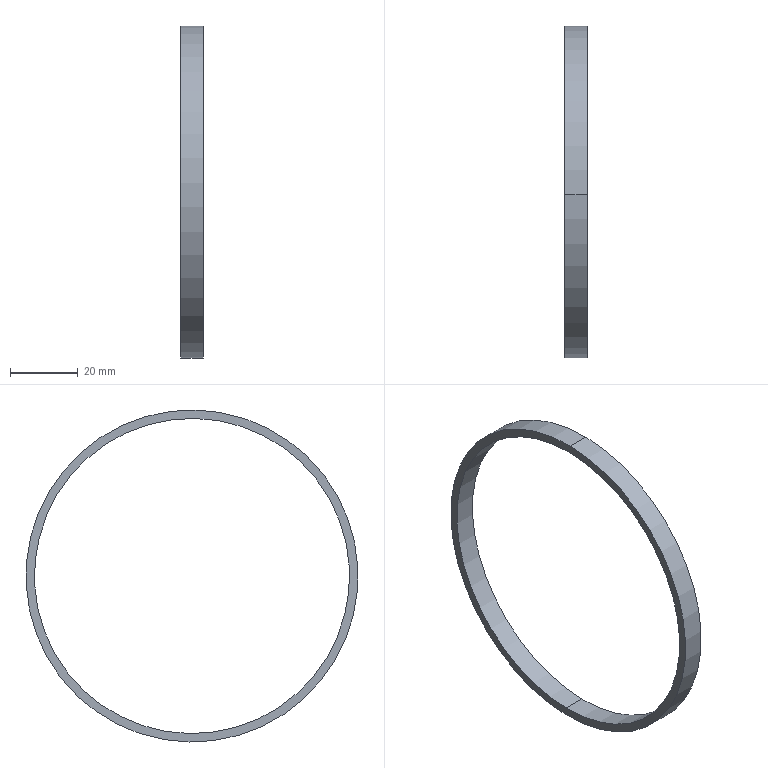Component | SolidWorks | 216InnerTubeAssembly-1_RetainingRing-1 | 1 solid | 6 faces | box 6.5 x 98 x 98 mm | volume 4875 mm3 | cylinder 4 | plane 2 | commonest cylinder face diameters 98 x2 93 x2 | material Alloy Steel
build123d program:
from build123d import *

# Parameters (mm, degrees)
MODEL_W = 6.5
MODEL_H = 2.5


with BuildPart() as part:
    # Model → Revolve1 (revolve)
    with BuildSketch(Plane.XY, mode=Mode.PRIVATE) as revolve1_sk:
        with Locations((3.25, 47.75)):
            Rectangle(MODEL_W, MODEL_H)
    revolve(revolve1_sk.sketch.rotate(Axis((0, 0, 0), (1, 0, 0)), 90), axis=Axis((0, 0, 0), (1, 0, 0)))


solid = part.part

# Placed as in the assembly
solid = solid.moved(Location((2893.278, 0, 0), (0, 0, 0)))
STEP:
#1=CARTESIAN_POINT('',(114.164,-0.03464,1.929));
#2=VERTEX_POINT('',#1);
#3=CARTESIAN_POINT('',(114.164,0.03464,-1.929));
#4=VERTEX_POINT('',#3);
#5=CARTESIAN_POINT('',(114.164,-0.,0.));
#6=DIRECTION('',(-1.,-0.,0.));
#7=DIRECTION('',(0.,-0.01796,0.9998));
#8=AXIS2_PLACEMENT_3D('',#5,#6,#7);
#9=CIRCLE('',#8,1.929);
#10=EDGE_CURVE('',#2,#4,#9,.T.);
#11=ORIENTED_EDGE('',*,*,#10,.T.);
#12=CARTESIAN_POINT('',(113.909,0.03464,-1.929));
#13=VERTEX_POINT('',#12);
#14=CARTESIAN_POINT('',(113.909,0.03464,-1.929));
#15=DIRECTION('',(-1.,-0.,0.));
#16=VECTOR('',#15,39.37);
#17=LINE('',#14,#16);
#18=EDGE_CURVE('',#4,#13,#17,.T.);
#19=ORIENTED_EDGE('',*,*,#18,.T.);
#20=CARTESIAN_POINT('',(113.909,-0.03464,1.929));
#21=VERTEX_POINT('',#20);
#22=CARTESIAN_POINT('',(113.909,-0.,0.));
#23=DIRECTION('',(-1.,-0.,0.));
#24=DIRECTION('',(0.,-0.01796,0.9998));
#25=AXIS2_PLACEMENT_3D('',#22,#23,#24);
#26=CIRCLE('',#25,1.929);
#27=EDGE_CURVE('',#21,#13,#26,.T.);
#28=ORIENTED_EDGE('',*,*,#27,.F.);
#29=CARTESIAN_POINT('',(113.909,-0.03464,1.929));
#30=DIRECTION('',(-1.,-0.,0.));
#31=VECTOR('',#30,39.37);
#32=LINE('',#29,#31);
#33=EDGE_CURVE('',#2,#21,#32,.T.);
#34=ORIENTED_EDGE('',*,*,#33,.F.);
#35=EDGE_LOOP('',(#11,#19,#28,#34));
#36=FACE_OUTER_BOUND('',#35,.T.);
#37=CARTESIAN_POINT('',(113.909,-0.,0.));
#38=DIRECTION('',(-1.,-0.,0.));
#39=DIRECTION('',(0.,-0.01796,0.9998));
#40=AXIS2_PLACEMENT_3D('',#37,#38,#39);
#41=CYLINDRICAL_SURFACE('',#40,1.929);
#42=ADVANCED_FACE('',(#36),#41,.T.);
#43=CARTESIAN_POINT('',(114.164,0.03287,-1.83));
#44=VERTEX_POINT('',#43);
#45=CARTESIAN_POINT('',(114.164,-0.03287,1.83));
#46=VERTEX_POINT('',#45);
#47=CARTESIAN_POINT('',(114.164,-0.,0.));
#48=DIRECTION('',(-1.,-0.,0.));
#49=DIRECTION('',(0.,-0.01796,0.9998));
#50=AXIS2_PLACEMENT_3D('',#47,#48,#49);
#51=CIRCLE('',#50,1.831);
#52=EDGE_CURVE('',#44,#46,#51,.T.);
#53=ORIENTED_EDGE('',*,*,#52,.F.);
#54=CARTESIAN_POINT('',(113.909,0.03287,-1.83));
#55=VERTEX_POINT('',#54);
#56=CARTESIAN_POINT('',(113.909,0.03287,-1.83));
#57=DIRECTION('',(-1.,-0.,0.));
#58=VECTOR('',#57,39.37);
#59=LINE('',#56,#58);
#60=EDGE_CURVE('',#44,#55,#59,.T.);
#61=ORIENTED_EDGE('',*,*,#60,.T.);
#62=CARTESIAN_POINT('',(113.909,-0.03287,1.83));
#63=VERTEX_POINT('',#62);
#64=CARTESIAN_POINT('',(113.909,-0.,0.));
#65=DIRECTION('',(-1.,-0.,0.));
#66=DIRECTION('',(0.,-0.01796,0.9998));
#67=AXIS2_PLACEMENT_3D('',#64,#65,#66);
#68=CIRCLE('',#67,1.831);
#69=EDGE_CURVE('',#55,#63,#68,.T.);
#70=ORIENTED_EDGE('',*,*,#69,.T.);
#71=CARTESIAN_POINT('',(113.909,-0.03287,1.83));
#72=DIRECTION('',(-1.,-0.,0.));
#73=VECTOR('',#72,39.37);
#74=LINE('',#71,#73);
#75=EDGE_CURVE('',#46,#63,#74,.T.);
#76=ORIENTED_EDGE('',*,*,#75,.F.);
#77=EDGE_LOOP('',(#53,#61,#70,#76));
#78=FACE_OUTER_BOUND('',#77,.T.);
#79=CARTESIAN_POINT('',(113.909,-0.,0.));
#80=DIRECTION('',(-1.,-0.,0.));
#81=DIRECTION('',(0.,-0.01796,0.9998));
#82=AXIS2_PLACEMENT_3D('',#79,#80,#81);
#83=CYLINDRICAL_SURFACE('',#82,1.831);
#84=ADVANCED_FACE('',(#78),#83,.F.);
#85=ORIENTED_EDGE('',*,*,#10,.F.);
#86=CARTESIAN_POINT('',(114.164,-0.,0.));
#87=DIRECTION('',(-1.,-0.,0.));
#88=DIRECTION('',(0.,-0.01796,0.9998));
#89=AXIS2_PLACEMENT_3D('',#86,#87,#88);
#90=CIRCLE('',#89,1.929);
#91=EDGE_CURVE('',#4,#2,#90,.T.);
#92=ORIENTED_EDGE('',*,*,#91,.F.);
#93=EDGE_LOOP('',(#85,#92));
#94=FACE_OUTER_BOUND('',#93,.T.);
#95=CARTESIAN_POINT('',(114.164,-0.,0.));
#96=DIRECTION('',(-1.,-0.,0.));
#97=DIRECTION('',(0.,-0.01796,0.9998));
#98=AXIS2_PLACEMENT_3D('',#95,#96,#97);
#99=CIRCLE('',#98,1.831);
#100=EDGE_CURVE('',#46,#44,#99,.T.);
#101=ORIENTED_EDGE('',*,*,#100,.T.);
#102=ORIENTED_EDGE('',*,*,#52,.T.);
#103=EDGE_LOOP('',(#101,#102));
#104=FACE_BOUND('',#103,.T.);
#105=CARTESIAN_POINT('',(114.164,1.929,0.03464));
#106=DIRECTION('',(-1.,-0.,0.));
#107=DIRECTION('',(0.,-0.01796,0.9998));
#108=AXIS2_PLACEMENT_3D('',#105,#106,#107);
#109=PLANE('',#108);
#110=ADVANCED_FACE('',(#94,#104),#109,.F.);
#111=ORIENTED_EDGE('',*,*,#60,.F.);
#112=ORIENTED_EDGE('',*,*,#100,.F.);
#113=ORIENTED_EDGE('',*,*,#75,.T.);
#114=CARTESIAN_POINT('',(113.909,-0.,0.));
#115=DIRECTION('',(-1.,-0.,0.));
#116=DIRECTION('',(0.,-0.01796,0.9998));
#117=AXIS2_PLACEMENT_3D('',#114,#115,#116);
#118=CIRCLE('',#117,1.831);
#119=EDGE_CURVE('',#63,#55,#118,.T.);
#120=ORIENTED_EDGE('',*,*,#119,.T.);
#121=EDGE_LOOP('',(#111,#112,#113,#120));
#122=FACE_OUTER_BOUND('',#121,.T.);
#123=CARTESIAN_POINT('',(113.909,-0.,0.));
#124=DIRECTION('',(-1.,-0.,0.));
#125=DIRECTION('',(0.,-0.01796,0.9998));
#126=AXIS2_PLACEMENT_3D('',#123,#124,#125);
#127=CYLINDRICAL_SURFACE('',#126,1.831);
#128=ADVANCED_FACE('',(#122),#127,.F.);
#129=ORIENTED_EDGE('',*,*,#119,.F.);
#130=ORIENTED_EDGE('',*,*,#69,.F.);
#131=EDGE_LOOP('',(#129,#130));
#132=FACE_BOUND('',#131,.T.);
#133=ORIENTED_EDGE('',*,*,#27,.T.);
#134=CARTESIAN_POINT('',(113.909,-0.,0.));
#135=DIRECTION('',(-1.,-0.,0.));
#136=DIRECTION('',(0.,-0.01796,0.9998));
#137=AXIS2_PLACEMENT_3D('',#134,#135,#136);
#138=CIRCLE('',#137,1.929);
#139=EDGE_CURVE('',#13,#21,#138,.T.);
#140=ORIENTED_EDGE('',*,*,#139,.T.);
#141=EDGE_LOOP('',(#133,#140));
#142=FACE_OUTER_BOUND('',#141,.T.);
#143=CARTESIAN_POINT('',(113.909,1.929,0.03464));
#144=DIRECTION('',(1.,0.,-0.));
#145=DIRECTION('',(-0.,0.01796,-0.9998));
#146=AXIS2_PLACEMENT_3D('',#143,#144,#145);
#147=PLANE('',#146);
#148=ADVANCED_FACE('',(#132,#142),#147,.F.);
#149=ORIENTED_EDGE('',*,*,#18,.F.);
#150=ORIENTED_EDGE('',*,*,#91,.T.);
#151=ORIENTED_EDGE('',*,*,#33,.T.);
#152=ORIENTED_EDGE('',*,*,#139,.F.);
#153=EDGE_LOOP('',(#149,#150,#151,#152));
#154=FACE_OUTER_BOUND('',#153,.T.);
#155=CARTESIAN_POINT('',(113.909,-0.,0.));
#156=DIRECTION('',(-1.,-0.,0.));
#157=DIRECTION('',(0.,-0.01796,0.9998));
#158=AXIS2_PLACEMENT_3D('',#155,#156,#157);
#159=CYLINDRICAL_SURFACE('',#158,1.929);
#160=ADVANCED_FACE('',(#154),#159,.T.);
#161=CLOSED_SHELL('',(#42,#84,#110,#128,#148,#160));
#162=MANIFOLD_SOLID_BREP('',#161);
#163=CARTESIAN_POINT('',(0.,0.,0.));
#164=DIRECTION('',(0.,0.,1.));
#165=DIRECTION('',(1.,0.,0.));
#166=AXIS2_PLACEMENT_3D('',#163,#164,#165);
#167=(LENGTH_UNIT()NAMED_UNIT(*)SI_UNIT($,.METRE.));
#168=LENGTH_MEASURE_WITH_UNIT(LENGTH_MEASURE(0.0254),#167);
#169=DIMENSIONAL_EXPONENTS(1.,0.,0.,0.,0.,0.,0.);
#170=(CONVERSION_BASED_UNIT('',#168)LENGTH_UNIT()NAMED_UNIT(#169));
#171=UNCERTAINTY_MEASURE_WITH_UNIT(LENGTH_MEASURE(0.00001),#170,'','');
#172=(NAMED_UNIT(*)PLANE_ANGLE_UNIT()SI_UNIT($,.RADIAN.));
#173=(NAMED_UNIT(*)SI_UNIT($,.STERADIAN.)SOLID_ANGLE_UNIT());
#174=(GEOMETRIC_REPRESENTATION_CONTEXT(3)GLOBAL_UNCERTAINTY_ASSIGNED_CONTEXT((#171))GLOBAL_UNIT_ASSIGNED_CONTEXT((#170,#172,#173))REPRESENTATION_CONTEXT('',''));
#175=ADVANCED_BREP_SHAPE_REPRESENTATION('',(#162,#166),#174);
#176=COLOUR_RGB('',0.7922,0.8196,0.9333);
#177=FILL_AREA_STYLE_COLOUR('',#176);
#178=FILL_AREA_STYLE('',(#177));
#179=SURFACE_STYLE_FILL_AREA(#178);
#180=SURFACE_SIDE_STYLE('',(#179));
#181=SURFACE_STYLE_USAGE(.BOTH.,#180);
#182=PRESENTATION_STYLE_ASSIGNMENT((#181));
#183=STYLED_ITEM('',(#182),#162);
#184=(LENGTH_UNIT()NAMED_UNIT(*)SI_UNIT($,.METRE.));
#185=LENGTH_MEASURE_WITH_UNIT(LENGTH_MEASURE(0.0254),#184);
#186=DIMENSIONAL_EXPONENTS(1.,0.,0.,0.,0.,0.,0.);
#187=(CONVERSION_BASED_UNIT('',#185)LENGTH_UNIT()NAMED_UNIT(#186));
#188=UNCERTAINTY_MEASURE_WITH_UNIT(LENGTH_MEASURE(0.00001),#187,'','');
#189=(NAMED_UNIT(*)PLANE_ANGLE_UNIT()SI_UNIT($,.RADIAN.));
#190=(NAMED_UNIT(*)SI_UNIT($,.STERADIAN.)SOLID_ANGLE_UNIT());
#191=(GEOMETRIC_REPRESENTATION_CONTEXT(3)GLOBAL_UNCERTAINTY_ASSIGNED_CONTEXT((#188))GLOBAL_UNIT_ASSIGNED_CONTEXT((#187,#189,#190))REPRESENTATION_CONTEXT('',''));
#192=MECHANICAL_DESIGN_GEOMETRIC_PRESENTATION_REPRESENTATION('',(#183),#191);
#193=PRESENTATION_LAYER_ASSIGNMENT('','',(#183));